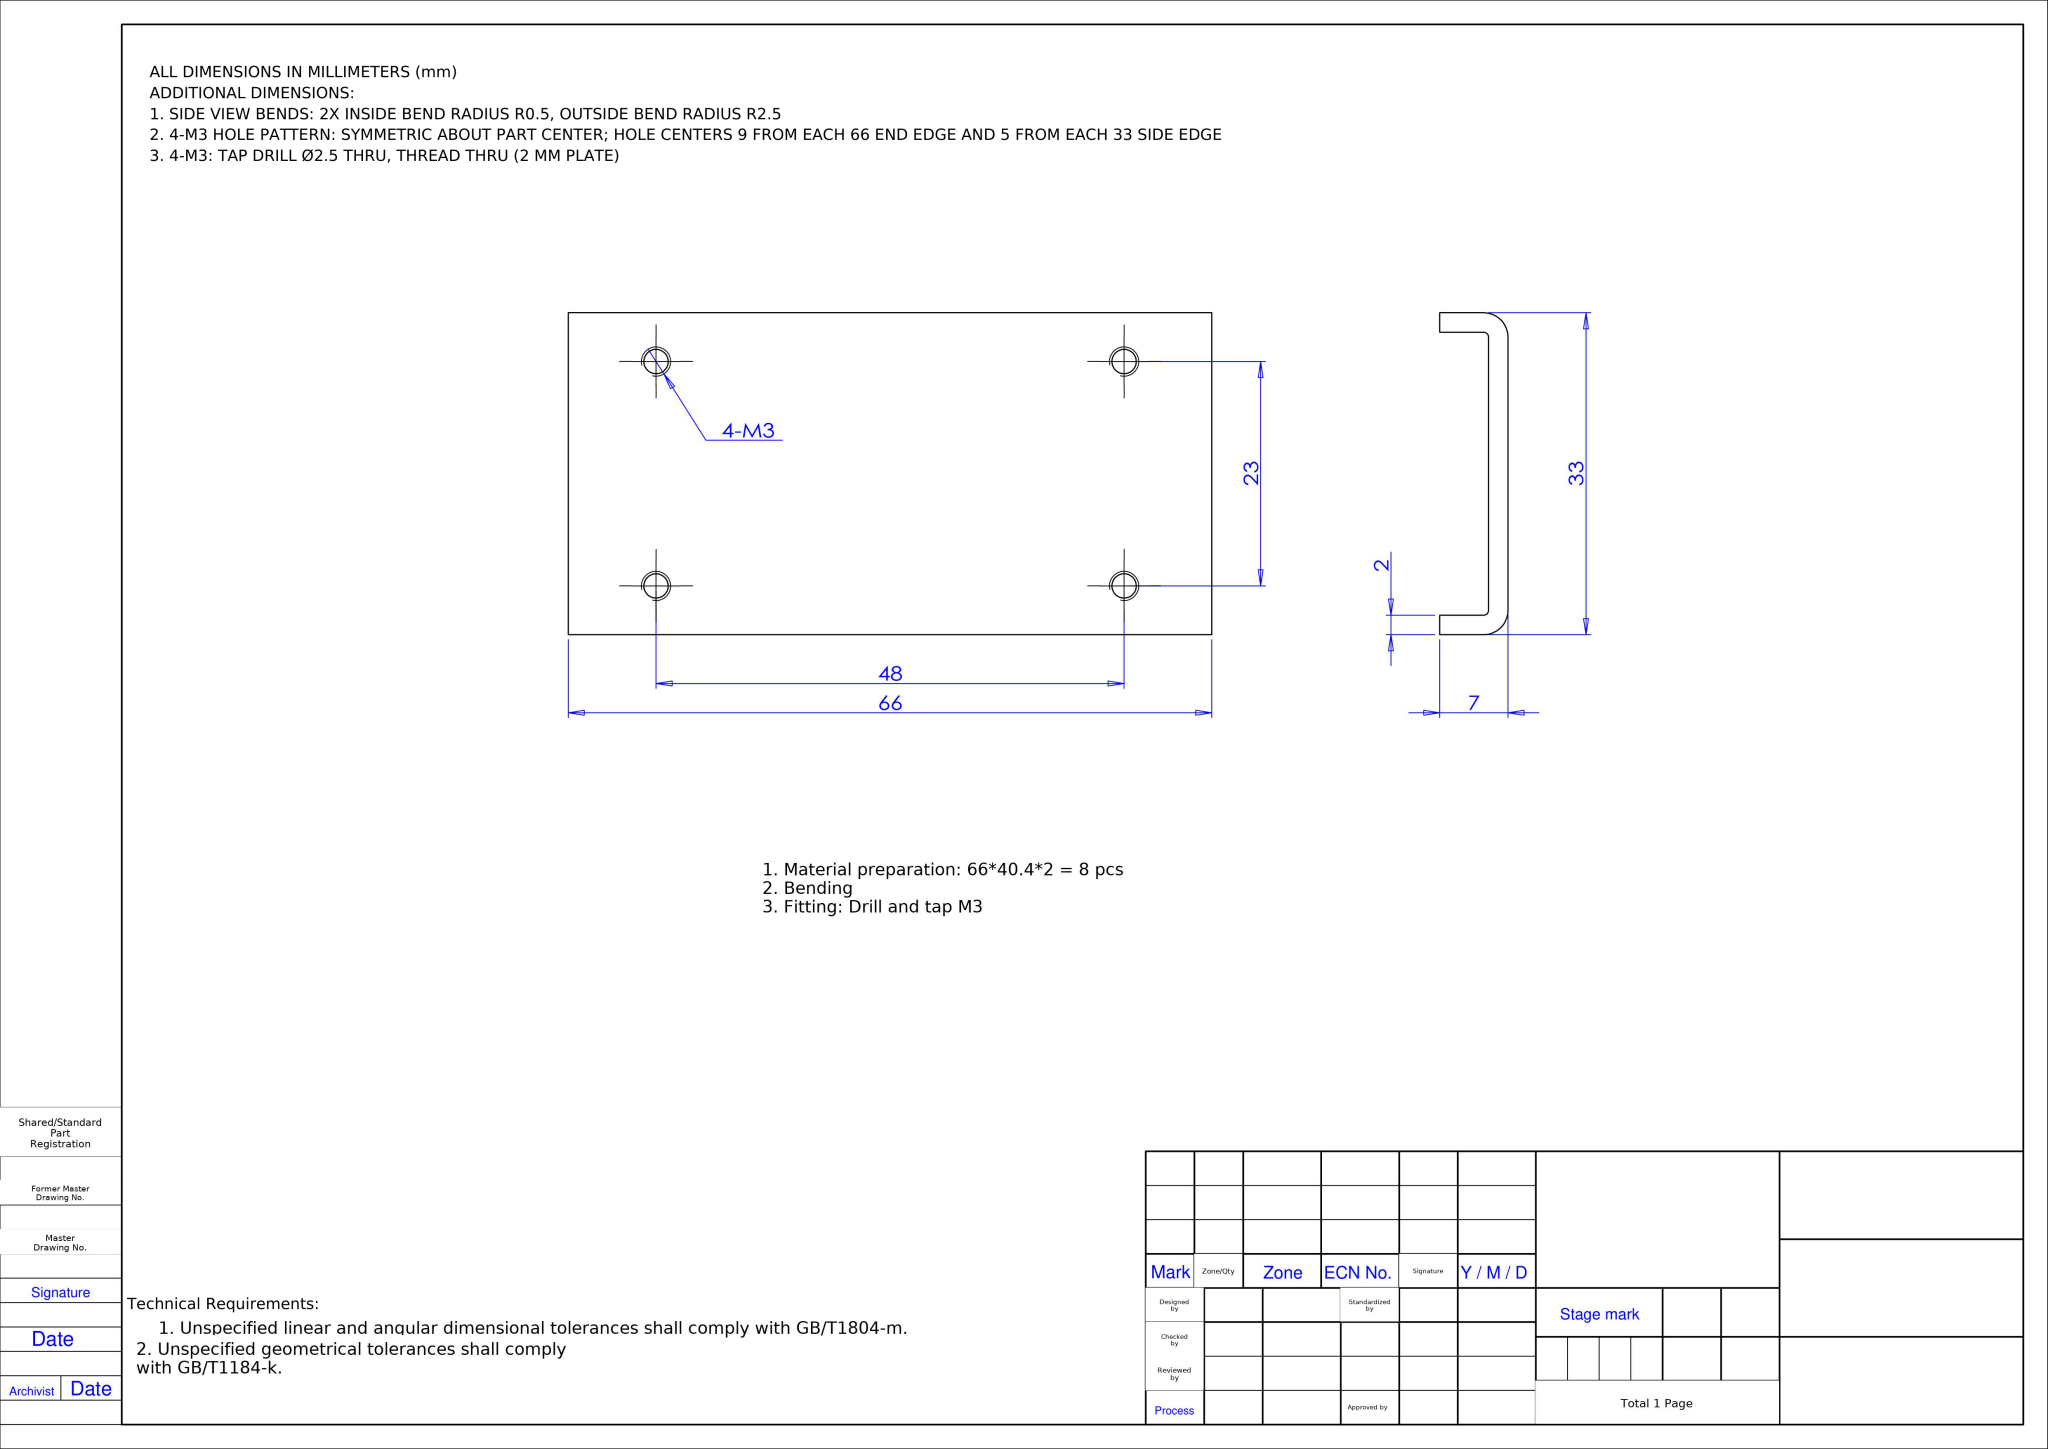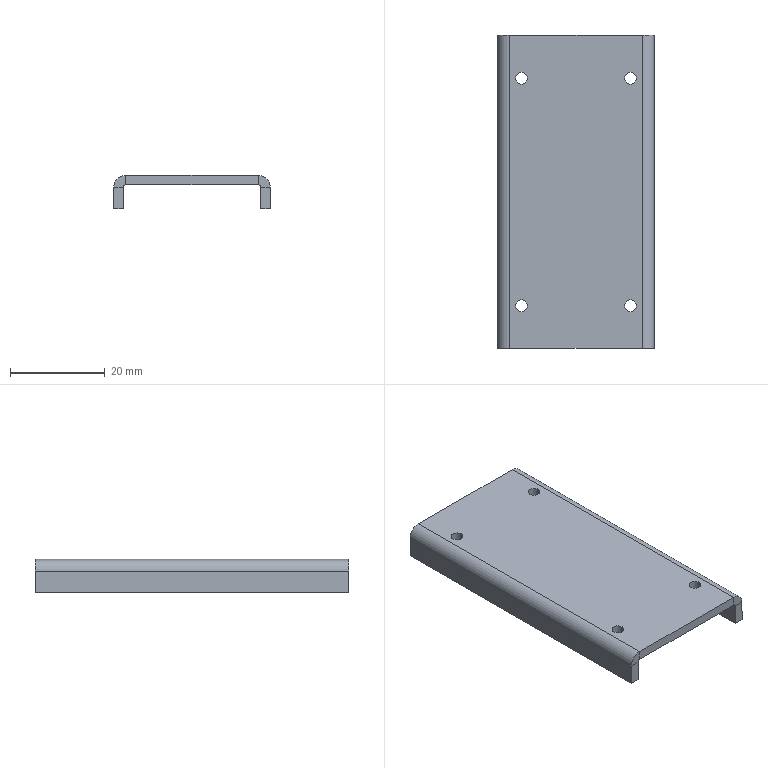Part | NX | mm | 1 solid | 30 faces | box 33 x 66 x 7 mm | volume 5467 mm3 | plane 18 | cylinder 12 | commonest cylinder face diameters 2.5 x8 5 x2 1 x2